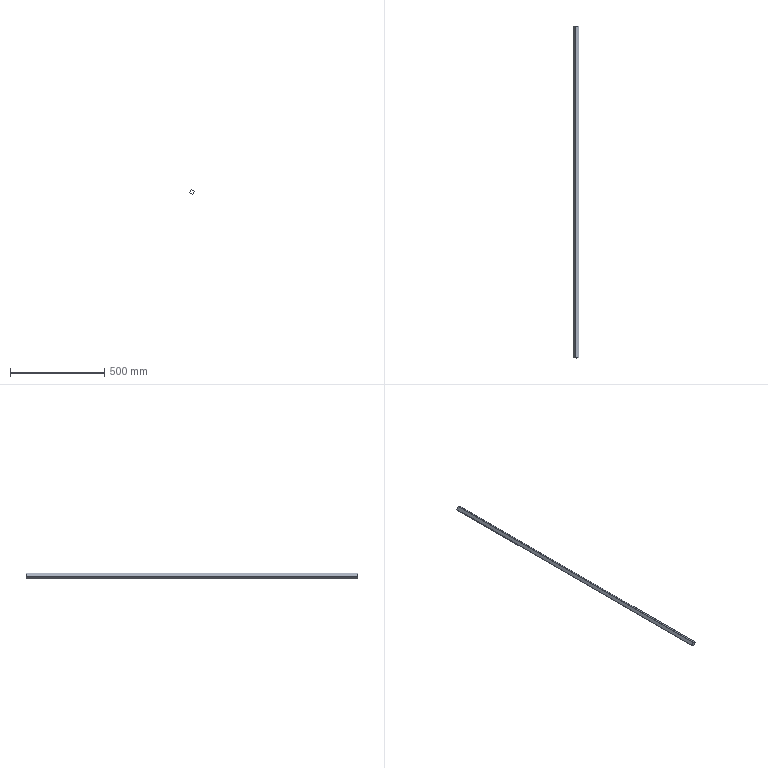Component | SolidWorks | FrontDoorFlangeWelding-2_FrontDoorRectangularTubeFrameWelding-1_1760RectangularTube-1 | 1 solid | 10 faces | box 27.3 x 1760 x 27.3 mm | volume 133760 mm3 | plane 10
STEP:
#1=CARTESIAN_POINT('',(1.932,32.798,54.983));
#2=VERTEX_POINT('',#1);
#3=CARTESIAN_POINT('',(1.54,32.798,54.3));
#4=VERTEX_POINT('',#3);
#5=CARTESIAN_POINT('',(1.932,32.798,54.983));
#6=DIRECTION('',(-0.4971,0.,-0.8677));
#7=VECTOR('',#6,39.37);
#8=LINE('',#5,#7);
#9=EDGE_CURVE('',#2,#4,#8,.T.);
#10=ORIENTED_EDGE('',*,*,#9,.T.);
#11=CARTESIAN_POINT('',(0.8573,32.798,54.691));
#12=VERTEX_POINT('',#11);
#13=CARTESIAN_POINT('',(1.54,32.798,54.3));
#14=DIRECTION('',(-0.8677,-0.,0.4971));
#15=VECTOR('',#14,39.37);
#16=LINE('',#13,#15);
#17=EDGE_CURVE('',#4,#12,#16,.T.);
#18=ORIENTED_EDGE('',*,*,#17,.T.);
#19=CARTESIAN_POINT('',(1.249,32.798,55.374));
#20=VERTEX_POINT('',#19);
#21=CARTESIAN_POINT('',(1.249,32.798,55.374));
#22=DIRECTION('',(0.4971,-0.,0.8677));
#23=VECTOR('',#22,39.37);
#24=LINE('',#21,#23);
#25=EDGE_CURVE('',#12,#20,#24,.T.);
#26=ORIENTED_EDGE('',*,*,#25,.T.);
#27=CARTESIAN_POINT('',(1.932,32.798,54.983));
#28=DIRECTION('',(0.8677,0.,-0.4971));
#29=VECTOR('',#28,39.37);
#30=LINE('',#27,#29);
#31=EDGE_CURVE('',#20,#2,#30,.T.);
#32=ORIENTED_EDGE('',*,*,#31,.T.);
#33=EDGE_LOOP('',(#10,#18,#26,#32));
#34=FACE_OUTER_BOUND('',#33,.T.);
#35=CARTESIAN_POINT('',(1.526,32.798,54.353));
#36=VERTEX_POINT('',#35);
#37=CARTESIAN_POINT('',(0.911,32.798,54.706));
#38=VERTEX_POINT('',#37);
#39=CARTESIAN_POINT('',(1.526,32.798,54.353));
#40=DIRECTION('',(-0.8677,-0.,0.4971));
#41=VECTOR('',#40,39.37);
#42=LINE('',#39,#41);
#43=EDGE_CURVE('',#36,#38,#42,.T.);
#44=ORIENTED_EDGE('',*,*,#43,.F.);
#45=CARTESIAN_POINT('',(1.878,32.798,54.968));
#46=VERTEX_POINT('',#45);
#47=CARTESIAN_POINT('',(1.878,32.798,54.968));
#48=DIRECTION('',(-0.4971,0.,-0.8677));
#49=VECTOR('',#48,39.37);
#50=LINE('',#47,#49);
#51=EDGE_CURVE('',#46,#36,#50,.T.);
#52=ORIENTED_EDGE('',*,*,#51,.F.);
#53=CARTESIAN_POINT('',(1.263,32.798,55.32));
#54=VERTEX_POINT('',#53);
#55=CARTESIAN_POINT('',(1.878,32.798,54.968));
#56=DIRECTION('',(0.8677,0.,-0.4971));
#57=VECTOR('',#56,39.37);
#58=LINE('',#55,#57);
#59=EDGE_CURVE('',#54,#46,#58,.T.);
#60=ORIENTED_EDGE('',*,*,#59,.F.);
#61=CARTESIAN_POINT('',(1.263,32.798,55.32));
#62=DIRECTION('',(0.4971,-0.,0.8677));
#63=VECTOR('',#62,39.37);
#64=LINE('',#61,#63);
#65=EDGE_CURVE('',#38,#54,#64,.T.);
#66=ORIENTED_EDGE('',*,*,#65,.F.);
#67=EDGE_LOOP('',(#44,#52,#60,#66));
#68=FACE_BOUND('',#67,.T.);
#69=CARTESIAN_POINT('',(-0.516,32.798,54.687));
#70=DIRECTION('',(-0.,1.,0.));
#71=DIRECTION('',(-0.8677,-0.,0.4971));
#72=AXIS2_PLACEMENT_3D('',#69,#70,#71);
#73=PLANE('',#72);
#74=ADVANCED_FACE('',(#34,#68),#73,.T.);
#75=CARTESIAN_POINT('',(1.932,-36.493,54.983));
#76=VERTEX_POINT('',#75);
#77=CARTESIAN_POINT('',(1.54,-36.493,54.3));
#78=VERTEX_POINT('',#77);
#79=CARTESIAN_POINT('',(1.932,-36.493,54.983));
#80=DIRECTION('',(-0.4971,0.,-0.8677));
#81=VECTOR('',#80,39.37);
#82=LINE('',#79,#81);
#83=EDGE_CURVE('',#76,#78,#82,.T.);
#84=ORIENTED_EDGE('',*,*,#83,.F.);
#85=CARTESIAN_POINT('',(1.249,-36.493,55.374));
#86=VERTEX_POINT('',#85);
#87=CARTESIAN_POINT('',(1.932,-36.493,54.983));
#88=DIRECTION('',(0.8677,0.,-0.4971));
#89=VECTOR('',#88,39.37);
#90=LINE('',#87,#89);
#91=EDGE_CURVE('',#86,#76,#90,.T.);
#92=ORIENTED_EDGE('',*,*,#91,.F.);
#93=CARTESIAN_POINT('',(0.8573,-36.493,54.691));
#94=VERTEX_POINT('',#93);
#95=CARTESIAN_POINT('',(1.249,-36.493,55.374));
#96=DIRECTION('',(0.4971,-0.,0.8677));
#97=VECTOR('',#96,39.37);
#98=LINE('',#95,#97);
#99=EDGE_CURVE('',#94,#86,#98,.T.);
#100=ORIENTED_EDGE('',*,*,#99,.F.);
#101=CARTESIAN_POINT('',(1.54,-36.493,54.3));
#102=DIRECTION('',(-0.8677,-0.,0.4971));
#103=VECTOR('',#102,39.37);
#104=LINE('',#101,#103);
#105=EDGE_CURVE('',#78,#94,#104,.T.);
#106=ORIENTED_EDGE('',*,*,#105,.F.);
#107=EDGE_LOOP('',(#84,#92,#100,#106));
#108=FACE_OUTER_BOUND('',#107,.T.);
#109=CARTESIAN_POINT('',(1.878,-36.493,54.968));
#110=VERTEX_POINT('',#109);
#111=CARTESIAN_POINT('',(1.526,-36.493,54.353));
#112=VERTEX_POINT('',#111);
#113=CARTESIAN_POINT('',(1.878,-36.493,54.968));
#114=DIRECTION('',(-0.4971,0.,-0.8677));
#115=VECTOR('',#114,39.37);
#116=LINE('',#113,#115);
#117=EDGE_CURVE('',#110,#112,#116,.T.);
#118=ORIENTED_EDGE('',*,*,#117,.T.);
#119=CARTESIAN_POINT('',(0.911,-36.493,54.706));
#120=VERTEX_POINT('',#119);
#121=CARTESIAN_POINT('',(1.526,-36.493,54.353));
#122=DIRECTION('',(-0.8677,-0.,0.4971));
#123=VECTOR('',#122,39.37);
#124=LINE('',#121,#123);
#125=EDGE_CURVE('',#112,#120,#124,.T.);
#126=ORIENTED_EDGE('',*,*,#125,.T.);
#127=CARTESIAN_POINT('',(1.263,-36.493,55.32));
#128=VERTEX_POINT('',#127);
#129=CARTESIAN_POINT('',(1.263,-36.493,55.32));
#130=DIRECTION('',(0.4971,-0.,0.8677));
#131=VECTOR('',#130,39.37);
#132=LINE('',#129,#131);
#133=EDGE_CURVE('',#120,#128,#132,.T.);
#134=ORIENTED_EDGE('',*,*,#133,.T.);
#135=CARTESIAN_POINT('',(1.878,-36.493,54.968));
#136=DIRECTION('',(0.8677,0.,-0.4971));
#137=VECTOR('',#136,39.37);
#138=LINE('',#135,#137);
#139=EDGE_CURVE('',#128,#110,#138,.T.);
#140=ORIENTED_EDGE('',*,*,#139,.T.);
#141=EDGE_LOOP('',(#118,#126,#134,#140));
#142=FACE_BOUND('',#141,.T.);
#143=CARTESIAN_POINT('',(-0.516,-36.493,54.687));
#144=DIRECTION('',(-0.,1.,0.));
#145=DIRECTION('',(-0.8677,-0.,0.4971));
#146=AXIS2_PLACEMENT_3D('',#143,#144,#145);
#147=PLANE('',#146);
#148=ADVANCED_FACE('',(#108,#142),#147,.F.);
#149=ORIENTED_EDGE('',*,*,#83,.T.);
#150=CARTESIAN_POINT('',(1.54,32.798,54.3));
#151=DIRECTION('',(0.,-1.,-0.));
#152=VECTOR('',#151,39.37);
#153=LINE('',#150,#152);
#154=EDGE_CURVE('',#4,#78,#153,.T.);
#155=ORIENTED_EDGE('',*,*,#154,.F.);
#156=ORIENTED_EDGE('',*,*,#9,.F.);
#157=CARTESIAN_POINT('',(1.932,32.798,54.983));
#158=DIRECTION('',(0.,-1.,-0.));
#159=VECTOR('',#158,39.37);
#160=LINE('',#157,#159);
#161=EDGE_CURVE('',#2,#76,#160,.T.);
#162=ORIENTED_EDGE('',*,*,#161,.T.);
#163=EDGE_LOOP('',(#149,#155,#156,#162));
#164=FACE_OUTER_BOUND('',#163,.T.);
#165=CARTESIAN_POINT('',(1.932,32.798,54.983));
#166=DIRECTION('',(-0.8677,-0.,0.4971));
#167=DIRECTION('',(0.4971,-0.,0.8677));
#168=AXIS2_PLACEMENT_3D('',#165,#166,#167);
#169=PLANE('',#168);
#170=ADVANCED_FACE('',(#164),#169,.F.);
#171=ORIENTED_EDGE('',*,*,#105,.T.);
#172=CARTESIAN_POINT('',(0.8573,32.798,54.691));
#173=DIRECTION('',(0.,-1.,-0.));
#174=VECTOR('',#173,39.37);
#175=LINE('',#172,#174);
#176=EDGE_CURVE('',#12,#94,#175,.T.);
#177=ORIENTED_EDGE('',*,*,#176,.F.);
#178=ORIENTED_EDGE('',*,*,#17,.F.);
#179=ORIENTED_EDGE('',*,*,#154,.T.);
#180=EDGE_LOOP('',(#171,#177,#178,#179));
#181=FACE_OUTER_BOUND('',#180,.T.);
#182=CARTESIAN_POINT('',(1.54,32.798,54.3));
#183=DIRECTION('',(0.4971,-0.,0.8677));
#184=DIRECTION('',(-0.,1.,0.));
#185=AXIS2_PLACEMENT_3D('',#182,#183,#184);
#186=PLANE('',#185);
#187=ADVANCED_FACE('',(#181),#186,.F.);
#188=ORIENTED_EDGE('',*,*,#99,.T.);
#189=CARTESIAN_POINT('',(1.249,32.798,55.374));
#190=DIRECTION('',(0.,-1.,-0.));
#191=VECTOR('',#190,39.37);
#192=LINE('',#189,#191);
#193=EDGE_CURVE('',#20,#86,#192,.T.);
#194=ORIENTED_EDGE('',*,*,#193,.F.);
#195=ORIENTED_EDGE('',*,*,#25,.F.);
#196=ORIENTED_EDGE('',*,*,#176,.T.);
#197=EDGE_LOOP('',(#188,#194,#195,#196));
#198=FACE_OUTER_BOUND('',#197,.T.);
#199=CARTESIAN_POINT('',(1.249,32.798,55.374));
#200=DIRECTION('',(0.8677,0.,-0.4971));
#201=DIRECTION('',(-0.4971,0.,-0.8677));
#202=AXIS2_PLACEMENT_3D('',#199,#200,#201);
#203=PLANE('',#202);
#204=ADVANCED_FACE('',(#198),#203,.F.);
#205=ORIENTED_EDGE('',*,*,#91,.T.);
#206=ORIENTED_EDGE('',*,*,#161,.F.);
#207=ORIENTED_EDGE('',*,*,#31,.F.);
#208=ORIENTED_EDGE('',*,*,#193,.T.);
#209=EDGE_LOOP('',(#205,#206,#207,#208));
#210=FACE_OUTER_BOUND('',#209,.T.);
#211=CARTESIAN_POINT('',(1.932,32.798,54.983));
#212=DIRECTION('',(-0.4971,0.,-0.8677));
#213=DIRECTION('',(0.,-1.,-0.));
#214=AXIS2_PLACEMENT_3D('',#211,#212,#213);
#215=PLANE('',#214);
#216=ADVANCED_FACE('',(#210),#215,.F.);
#217=ORIENTED_EDGE('',*,*,#117,.F.);
#218=CARTESIAN_POINT('',(1.878,32.798,54.968));
#219=DIRECTION('',(0.,-1.,-0.));
#220=VECTOR('',#219,39.37);
#221=LINE('',#218,#220);
#222=EDGE_CURVE('',#46,#110,#221,.T.);
#223=ORIENTED_EDGE('',*,*,#222,.F.);
#224=ORIENTED_EDGE('',*,*,#51,.T.);
#225=CARTESIAN_POINT('',(1.526,32.798,54.353));
#226=DIRECTION('',(0.,-1.,-0.));
#227=VECTOR('',#226,39.37);
#228=LINE('',#225,#227);
#229=EDGE_CURVE('',#36,#112,#228,.T.);
#230=ORIENTED_EDGE('',*,*,#229,.T.);
#231=EDGE_LOOP('',(#217,#223,#224,#230));
#232=FACE_OUTER_BOUND('',#231,.T.);
#233=CARTESIAN_POINT('',(1.878,32.798,54.968));
#234=DIRECTION('',(-0.8677,-0.,0.4971));
#235=DIRECTION('',(0.,-1.,-0.));
#236=AXIS2_PLACEMENT_3D('',#233,#234,#235);
#237=PLANE('',#236);
#238=ADVANCED_FACE('',(#232),#237,.T.);
#239=ORIENTED_EDGE('',*,*,#125,.F.);
#240=ORIENTED_EDGE('',*,*,#229,.F.);
#241=ORIENTED_EDGE('',*,*,#43,.T.);
#242=CARTESIAN_POINT('',(0.911,32.798,54.706));
#243=DIRECTION('',(0.,-1.,-0.));
#244=VECTOR('',#243,39.37);
#245=LINE('',#242,#244);
#246=EDGE_CURVE('',#38,#120,#245,.T.);
#247=ORIENTED_EDGE('',*,*,#246,.T.);
#248=EDGE_LOOP('',(#239,#240,#241,#247));
#249=FACE_OUTER_BOUND('',#248,.T.);
#250=CARTESIAN_POINT('',(1.526,32.798,54.353));
#251=DIRECTION('',(0.4971,-0.,0.8677));
#252=DIRECTION('',(-0.,1.,0.));
#253=AXIS2_PLACEMENT_3D('',#250,#251,#252);
#254=PLANE('',#253);
#255=ADVANCED_FACE('',(#249),#254,.T.);
#256=ORIENTED_EDGE('',*,*,#133,.F.);
#257=ORIENTED_EDGE('',*,*,#246,.F.);
#258=ORIENTED_EDGE('',*,*,#65,.T.);
#259=CARTESIAN_POINT('',(1.263,32.798,55.32));
#260=DIRECTION('',(0.,-1.,-0.));
#261=VECTOR('',#260,39.37);
#262=LINE('',#259,#261);
#263=EDGE_CURVE('',#54,#128,#262,.T.);
#264=ORIENTED_EDGE('',*,*,#263,.T.);
#265=EDGE_LOOP('',(#256,#257,#258,#264));
#266=FACE_OUTER_BOUND('',#265,.T.);
#267=CARTESIAN_POINT('',(1.263,32.798,55.32));
#268=DIRECTION('',(0.8677,0.,-0.4971));
#269=DIRECTION('',(-0.,1.,0.));
#270=AXIS2_PLACEMENT_3D('',#267,#268,#269);
#271=PLANE('',#270);
#272=ADVANCED_FACE('',(#266),#271,.T.);
#273=ORIENTED_EDGE('',*,*,#139,.F.);
#274=ORIENTED_EDGE('',*,*,#263,.F.);
#275=ORIENTED_EDGE('',*,*,#59,.T.);
#276=ORIENTED_EDGE('',*,*,#222,.T.);
#277=EDGE_LOOP('',(#273,#274,#275,#276));
#278=FACE_OUTER_BOUND('',#277,.T.);
#279=CARTESIAN_POINT('',(1.878,32.798,54.968));
#280=DIRECTION('',(-0.4971,0.,-0.8677));
#281=DIRECTION('',(0.,-1.,-0.));
#282=AXIS2_PLACEMENT_3D('',#279,#280,#281);
#283=PLANE('',#282);
#284=ADVANCED_FACE('',(#278),#283,.T.);
#285=CLOSED_SHELL('',(#74,#148,#170,#187,#204,#216,#238,#255,#272,#284));
#286=MANIFOLD_SOLID_BREP('',#285);
#287=CARTESIAN_POINT('',(0.,0.,0.));
#288=DIRECTION('',(0.,0.,1.));
#289=DIRECTION('',(1.,0.,0.));
#290=AXIS2_PLACEMENT_3D('',#287,#288,#289);
#291=(LENGTH_UNIT()NAMED_UNIT(*)SI_UNIT($,.METRE.));
#292=LENGTH_MEASURE_WITH_UNIT(LENGTH_MEASURE(0.0254),#291);
#293=DIMENSIONAL_EXPONENTS(1.,0.,0.,0.,0.,0.,0.);
#294=(CONVERSION_BASED_UNIT('',#292)LENGTH_UNIT()NAMED_UNIT(#293));
#295=UNCERTAINTY_MEASURE_WITH_UNIT(LENGTH_MEASURE(0.00001),#294,'','');
#296=(NAMED_UNIT(*)PLANE_ANGLE_UNIT()SI_UNIT($,.RADIAN.));
#297=(NAMED_UNIT(*)SI_UNIT($,.STERADIAN.)SOLID_ANGLE_UNIT());
#298=(GEOMETRIC_REPRESENTATION_CONTEXT(3)GLOBAL_UNCERTAINTY_ASSIGNED_CONTEXT((#295))GLOBAL_UNIT_ASSIGNED_CONTEXT((#294,#296,#297))REPRESENTATION_CONTEXT('',''));
#299=ADVANCED_BREP_SHAPE_REPRESENTATION('',(#286,#290),#298);
#300=COLOUR_RGB('',0.7922,0.8196,0.9333);
#301=FILL_AREA_STYLE_COLOUR('',#300);
#302=FILL_AREA_STYLE('',(#301));
#303=SURFACE_STYLE_FILL_AREA(#302);
#304=SURFACE_SIDE_STYLE('',(#303));
#305=SURFACE_STYLE_USAGE(.BOTH.,#304);
#306=PRESENTATION_STYLE_ASSIGNMENT((#305));
#307=STYLED_ITEM('',(#306),#286);
#308=PRESENTATION_LAYER_ASSIGNMENT('','',(#307));
#309=(LENGTH_UNIT()NAMED_UNIT(*)SI_UNIT($,.METRE.));
#310=LENGTH_MEASURE_WITH_UNIT(LENGTH_MEASURE(0.0254),#309);
#311=DIMENSIONAL_EXPONENTS(1.,0.,0.,0.,0.,0.,0.);
#312=(CONVERSION_BASED_UNIT('',#310)LENGTH_UNIT()NAMED_UNIT(#311));
#313=UNCERTAINTY_MEASURE_WITH_UNIT(LENGTH_MEASURE(0.00001),#312,'','');
#314=(NAMED_UNIT(*)PLANE_ANGLE_UNIT()SI_UNIT($,.RADIAN.));
#315=(NAMED_UNIT(*)SI_UNIT($,.STERADIAN.)SOLID_ANGLE_UNIT());
#316=(GEOMETRIC_REPRESENTATION_CONTEXT(3)GLOBAL_UNCERTAINTY_ASSIGNED_CONTEXT((#313))GLOBAL_UNIT_ASSIGNED_CONTEXT((#312,#314,#315))REPRESENTATION_CONTEXT('',''));
#317=MECHANICAL_DESIGN_GEOMETRIC_PRESENTATION_REPRESENTATION('',(#307),#316);